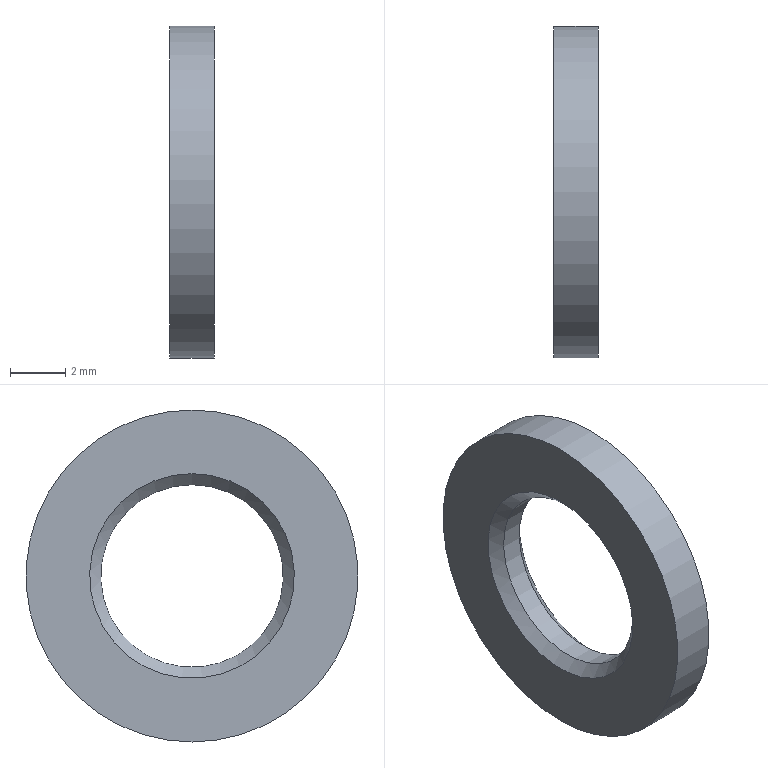Component | NX | WASHER_M6 | 1 solid | 6 faces | box 1.6 x 12 x 12 mm | volume 123 mm3 | cylinder 2 | plane 2 | cone 2 | commonest cylinder face diameters 12 x1 6.6 x1
STEP:
#1=CARTESIAN_POINT('',(0.,0.,0.));
#2=DIRECTION('',(0.,0.,1.));
#3=DIRECTION('',(1.,0.,0.));
#4=AXIS2_PLACEMENT_3D('',#1,#2,#3);
#5=CARTESIAN_POINT('',(10.307,66.5,-80.));
#6=VERTEX_POINT('',#5);
#7=CARTESIAN_POINT('',(10.307,66.5,-74.));
#8=DIRECTION('',(-1.,0.,0.));
#9=DIRECTION('',(0.,0.,-1.));
#10=AXIS2_PLACEMENT_3D('',#7,#8,#9);
#11=CIRCLE('',#10,6.);
#12=CARTESIAN_POINT('',(10.307,66.5,-74.));
#13=DIRECTION('',(-1.,0.,0.));
#14=DIRECTION('',(0.,0.,1.));
#15=AXIS2_PLACEMENT_3D('',#12,#13,#14);
#16=CYLINDRICAL_SURFACE('',#15,6.);
#17=CARTESIAN_POINT('',(3.142,0.));
#18=DIRECTION('',(1.,0.));
#19=VECTOR('',#18,1.);
#20=LINE('',#17,#19);
#21=(GEOMETRIC_REPRESENTATION_CONTEXT(2)PARAMETRIC_REPRESENTATION_CONTEXT()REPRESENTATION_CONTEXT('',''));
#22=DEFINITIONAL_REPRESENTATION('',(#20),#21);
#23=PCURVE('',#16,#22);
#24=CARTESIAN_POINT('',(10.307,66.5,-74.));
#25=DIRECTION('',(-1.,0.,0.));
#26=DIRECTION('',(0.,0.,1.));
#27=AXIS2_PLACEMENT_3D('',#24,#25,#26);
#28=PLANE('',#27);
#29=CARTESIAN_POINT('',(0.,0.));
#30=DIRECTION('',(-1.,0.));
#31=AXIS2_PLACEMENT_2D('',#29,#30);
#32=CIRCLE('',#31,6.);
#33=(GEOMETRIC_REPRESENTATION_CONTEXT(2)PARAMETRIC_REPRESENTATION_CONTEXT()REPRESENTATION_CONTEXT('',''));
#34=DEFINITIONAL_REPRESENTATION('',(#32),#33);
#35=PCURVE('',#28,#34);
#36=SURFACE_CURVE('',#11,(#23,#35),.PCURVE_S1.);
#37=EDGE_CURVE('',#6,#6,#36,.T.);
#38=ORIENTED_EDGE('',*,*,#37,.T.);
#39=CARTESIAN_POINT('',(8.707,66.5,-80.));
#40=VERTEX_POINT('',#39);
#41=CARTESIAN_POINT('',(10.307,66.5,-80.));
#42=CARTESIAN_POINT('',(8.707,66.5,-80.));
#43=B_SPLINE_CURVE_WITH_KNOTS('',1,(#41,#42),.UNSPECIFIED.,.F.,.F.,(2,2),(0.,1.6),.PIECEWISE_BEZIER_KNOTS.);
#44=CARTESIAN_POINT('',(9.425,0.));
#45=DIRECTION('',(0.,1.));
#46=VECTOR('',#45,1.);
#47=LINE('',#44,#46);
#48=(GEOMETRIC_REPRESENTATION_CONTEXT(2)PARAMETRIC_REPRESENTATION_CONTEXT()REPRESENTATION_CONTEXT('',''));
#49=DEFINITIONAL_REPRESENTATION('',(#47),#48);
#50=PCURVE('',#16,#49);
#51=CARTESIAN_POINT('',(3.142,0.));
#52=DIRECTION('',(0.,1.));
#53=VECTOR('',#52,1.);
#54=LINE('',#51,#53);
#55=(GEOMETRIC_REPRESENTATION_CONTEXT(2)PARAMETRIC_REPRESENTATION_CONTEXT()REPRESENTATION_CONTEXT('',''));
#56=DEFINITIONAL_REPRESENTATION('',(#54),#55);
#57=PCURVE('',#16,#56);
#58=SEAM_CURVE('',#43,(#50,#57),.PCURVE_S1.);
#59=EDGE_CURVE('',#6,#40,#58,.T.);
#60=ORIENTED_EDGE('',*,*,#59,.T.);
#61=CARTESIAN_POINT('',(8.707,66.5,-74.));
#62=DIRECTION('',(-1.,0.,0.));
#63=DIRECTION('',(0.,0.,-1.));
#64=AXIS2_PLACEMENT_3D('',#61,#62,#63);
#65=CIRCLE('',#64,6.);
#66=CARTESIAN_POINT('',(3.142,1.6));
#67=DIRECTION('',(1.,0.));
#68=VECTOR('',#67,1.);
#69=LINE('',#66,#68);
#70=(GEOMETRIC_REPRESENTATION_CONTEXT(2)PARAMETRIC_REPRESENTATION_CONTEXT()REPRESENTATION_CONTEXT('',''));
#71=DEFINITIONAL_REPRESENTATION('',(#69),#70);
#72=PCURVE('',#16,#71);
#73=CARTESIAN_POINT('',(8.707,66.5,-74.));
#74=DIRECTION('',(-1.,0.,0.));
#75=DIRECTION('',(0.,0.,1.));
#76=AXIS2_PLACEMENT_3D('',#73,#74,#75);
#77=PLANE('',#76);
#78=CARTESIAN_POINT('',(0.,0.));
#79=DIRECTION('',(-1.,0.));
#80=AXIS2_PLACEMENT_2D('',#78,#79);
#81=CIRCLE('',#80,6.);
#82=(GEOMETRIC_REPRESENTATION_CONTEXT(2)PARAMETRIC_REPRESENTATION_CONTEXT()REPRESENTATION_CONTEXT('',''));
#83=DEFINITIONAL_REPRESENTATION('',(#81),#82);
#84=PCURVE('',#77,#83);
#85=SURFACE_CURVE('',#65,(#72,#84),.PCURVE_S1.);
#86=EDGE_CURVE('',#40,#40,#85,.T.);
#87=ORIENTED_EDGE('',*,*,#86,.F.);
#88=ORIENTED_EDGE('',*,*,#59,.F.);
#89=EDGE_LOOP('',(#38,#60,#87,#88));
#90=FACE_BOUND('',#89,.T.);
#91=ADVANCED_FACE('',(#90),#16,.T.);
#92=CARTESIAN_POINT('',(9.907,66.5,-70.7));
#93=VERTEX_POINT('',#92);
#94=CARTESIAN_POINT('',(9.907,66.5,-74.));
#95=DIRECTION('',(1.,0.,0.));
#96=DIRECTION('',(0.,0.,1.));
#97=AXIS2_PLACEMENT_3D('',#94,#95,#96);
#98=CIRCLE('',#97,3.3);
#99=CARTESIAN_POINT('',(10.307,66.5,-74.));
#100=DIRECTION('',(-1.,0.,0.));
#101=DIRECTION('',(0.,0.,1.));
#102=AXIS2_PLACEMENT_3D('',#99,#100,#101);
#103=CYLINDRICAL_SURFACE('',#102,3.3);
#104=CARTESIAN_POINT('',(6.283,0.4));
#105=DIRECTION('',(-1.,0.));
#106=VECTOR('',#105,1.);
#107=LINE('',#104,#106);
#108=(GEOMETRIC_REPRESENTATION_CONTEXT(2)PARAMETRIC_REPRESENTATION_CONTEXT()REPRESENTATION_CONTEXT('',''));
#109=DEFINITIONAL_REPRESENTATION('',(#107),#108);
#110=PCURVE('',#103,#109);
#111=CARTESIAN_POINT('',(10.307,66.5,-74.));
#112=DIRECTION('',(1.,0.,0.));
#113=DIRECTION('',(0.,0.,-1.));
#114=AXIS2_PLACEMENT_3D('',#111,#112,#113);
#115=CONICAL_SURFACE('',#114,3.7,0.7854);
#116=CARTESIAN_POINT('',(3.142,-0.4));
#117=DIRECTION('',(1.,0.));
#118=VECTOR('',#117,1.);
#119=LINE('',#116,#118);
#120=(GEOMETRIC_REPRESENTATION_CONTEXT(2)PARAMETRIC_REPRESENTATION_CONTEXT()REPRESENTATION_CONTEXT('',''));
#121=DEFINITIONAL_REPRESENTATION('',(#119),#120);
#122=PCURVE('',#115,#121);
#123=SURFACE_CURVE('',#98,(#110,#122),.PCURVE_S1.);
#124=EDGE_CURVE('',#93,#93,#123,.T.);
#125=ORIENTED_EDGE('',*,*,#124,.F.);
#126=CARTESIAN_POINT('',(9.107,66.5,-70.7));
#127=VERTEX_POINT('',#126);
#128=CARTESIAN_POINT('',(9.907,66.5,-70.7));
#129=CARTESIAN_POINT('',(9.107,66.5,-70.7));
#130=B_SPLINE_CURVE_WITH_KNOTS('',1,(#128,#129),.UNSPECIFIED.,.F.,.F.,(2,2),(0.4,1.2),.PIECEWISE_BEZIER_KNOTS.);
#131=CARTESIAN_POINT('',(6.283,0.));
#132=DIRECTION('',(0.,1.));
#133=VECTOR('',#132,1.);
#134=LINE('',#131,#133);
#135=(GEOMETRIC_REPRESENTATION_CONTEXT(2)PARAMETRIC_REPRESENTATION_CONTEXT()REPRESENTATION_CONTEXT('',''));
#136=DEFINITIONAL_REPRESENTATION('',(#134),#135);
#137=PCURVE('',#103,#136);
#138=CARTESIAN_POINT('',(0.,0.));
#139=DIRECTION('',(0.,1.));
#140=VECTOR('',#139,1.);
#141=LINE('',#138,#140);
#142=(GEOMETRIC_REPRESENTATION_CONTEXT(2)PARAMETRIC_REPRESENTATION_CONTEXT()REPRESENTATION_CONTEXT('',''));
#143=DEFINITIONAL_REPRESENTATION('',(#141),#142);
#144=PCURVE('',#103,#143);
#145=SEAM_CURVE('',#130,(#137,#144),.PCURVE_S1.);
#146=EDGE_CURVE('',#93,#127,#145,.T.);
#147=ORIENTED_EDGE('',*,*,#146,.T.);
#148=CARTESIAN_POINT('',(9.107,66.5,-74.));
#149=DIRECTION('',(-1.,0.,0.));
#150=DIRECTION('',(0.,0.,1.));
#151=AXIS2_PLACEMENT_3D('',#148,#149,#150);
#152=CIRCLE('',#151,3.3);
#153=CARTESIAN_POINT('',(0.,1.2));
#154=DIRECTION('',(1.,0.));
#155=VECTOR('',#154,1.);
#156=LINE('',#153,#155);
#157=(GEOMETRIC_REPRESENTATION_CONTEXT(2)PARAMETRIC_REPRESENTATION_CONTEXT()REPRESENTATION_CONTEXT('',''));
#158=DEFINITIONAL_REPRESENTATION('',(#156),#157);
#159=PCURVE('',#103,#158);
#160=CARTESIAN_POINT('',(9.107,66.5,-74.));
#161=DIRECTION('',(-1.,0.,0.));
#162=DIRECTION('',(0.,0.,1.));
#163=AXIS2_PLACEMENT_3D('',#160,#161,#162);
#164=CONICAL_SURFACE('',#163,3.3,0.7854);
#165=CARTESIAN_POINT('',(0.,-0.));
#166=DIRECTION('',(1.,0.));
#167=VECTOR('',#166,1.);
#168=LINE('',#165,#167);
#169=(GEOMETRIC_REPRESENTATION_CONTEXT(2)PARAMETRIC_REPRESENTATION_CONTEXT()REPRESENTATION_CONTEXT('',''));
#170=DEFINITIONAL_REPRESENTATION('',(#168),#169);
#171=PCURVE('',#164,#170);
#172=SURFACE_CURVE('',#152,(#159,#171),.PCURVE_S1.);
#173=EDGE_CURVE('',#127,#127,#172,.T.);
#174=ORIENTED_EDGE('',*,*,#173,.F.);
#175=ORIENTED_EDGE('',*,*,#146,.F.);
#176=EDGE_LOOP('',(#125,#147,#174,#175));
#177=FACE_BOUND('',#176,.F.);
#178=ADVANCED_FACE('',(#177),#103,.F.);
#179=CARTESIAN_POINT('',(10.307,66.5,-70.3));
#180=VERTEX_POINT('',#179);
#181=CARTESIAN_POINT('',(10.307,66.5,-74.));
#182=DIRECTION('',(-1.,0.,0.));
#183=DIRECTION('',(0.,0.,1.));
#184=AXIS2_PLACEMENT_3D('',#181,#182,#183);
#185=CIRCLE('',#184,3.7);
#186=CARTESIAN_POINT('',(0.,0.));
#187=DIRECTION('',(1.,0.));
#188=AXIS2_PLACEMENT_2D('',#186,#187);
#189=CIRCLE('',#188,3.7);
#190=(GEOMETRIC_REPRESENTATION_CONTEXT(2)PARAMETRIC_REPRESENTATION_CONTEXT()REPRESENTATION_CONTEXT('',''));
#191=DEFINITIONAL_REPRESENTATION('',(#189),#190);
#192=PCURVE('',#28,#191);
#193=CARTESIAN_POINT('',(9.425,-0.));
#194=DIRECTION('',(-1.,0.));
#195=VECTOR('',#194,1.);
#196=LINE('',#193,#195);
#197=(GEOMETRIC_REPRESENTATION_CONTEXT(2)PARAMETRIC_REPRESENTATION_CONTEXT()REPRESENTATION_CONTEXT('',''));
#198=DEFINITIONAL_REPRESENTATION('',(#196),#197);
#199=PCURVE('',#115,#198);
#200=SURFACE_CURVE('',#185,(#192,#199),.PCURVE_S1.);
#201=EDGE_CURVE('',#180,#180,#200,.T.);
#202=ORIENTED_EDGE('',*,*,#201,.T.);
#203=EDGE_LOOP('',(#202));
#204=FACE_BOUND('',#203,.T.);
#205=ORIENTED_EDGE('',*,*,#37,.F.);
#206=EDGE_LOOP('',(#205));
#207=FACE_BOUND('',#206,.T.);
#208=ADVANCED_FACE('',(#204,#207),#28,.F.);
#209=CARTESIAN_POINT('',(8.707,66.5,-70.3));
#210=VERTEX_POINT('',#209);
#211=CARTESIAN_POINT('',(8.707,66.5,-74.));
#212=DIRECTION('',(1.,0.,0.));
#213=DIRECTION('',(0.,0.,1.));
#214=AXIS2_PLACEMENT_3D('',#211,#212,#213);
#215=CIRCLE('',#214,3.7);
#216=CARTESIAN_POINT('',(3.7,0.));
#217=CARTESIAN_POINT('',(3.7,-6.409));
#218=CARTESIAN_POINT('',(-1.85,-3.204));
#219=CARTESIAN_POINT('',(-7.4,-0.));
#220=CARTESIAN_POINT('',(-1.85,3.204));
#221=CARTESIAN_POINT('',(3.7,6.409));
#222=CARTESIAN_POINT('',(3.7,0.));
#223=(BOUNDED_CURVE()B_SPLINE_CURVE(2,(#216,#217,#218,#219,#220,#221,#222),.UNSPECIFIED.,.T.,.F.)B_SPLINE_CURVE_WITH_KNOTS((1,2,2,2,2,1),(-2.094,0.,2.094,4.189,6.283,8.378),.UNSPECIFIED.)CURVE()GEOMETRIC_REPRESENTATION_ITEM()RATIONAL_B_SPLINE_CURVE((1.,0.5,1.,0.5,1.,0.5,1.))REPRESENTATION_ITEM(''));
#224=(GEOMETRIC_REPRESENTATION_CONTEXT(2)PARAMETRIC_REPRESENTATION_CONTEXT()REPRESENTATION_CONTEXT('',''));
#225=DEFINITIONAL_REPRESENTATION('',(#223),#224);
#226=PCURVE('',#77,#225);
#227=CARTESIAN_POINT('',(6.283,0.4));
#228=DIRECTION('',(-1.,0.));
#229=VECTOR('',#228,1.);
#230=LINE('',#227,#229);
#231=(GEOMETRIC_REPRESENTATION_CONTEXT(2)PARAMETRIC_REPRESENTATION_CONTEXT()REPRESENTATION_CONTEXT('',''));
#232=DEFINITIONAL_REPRESENTATION('',(#230),#231);
#233=PCURVE('',#164,#232);
#234=SURFACE_CURVE('',#215,(#226,#233),.PCURVE_S1.);
#235=EDGE_CURVE('',#210,#210,#234,.T.);
#236=ORIENTED_EDGE('',*,*,#235,.T.);
#237=EDGE_LOOP('',(#236));
#238=FACE_BOUND('',#237,.T.);
#239=ORIENTED_EDGE('',*,*,#86,.T.);
#240=EDGE_LOOP('',(#239));
#241=FACE_BOUND('',#240,.T.);
#242=ADVANCED_FACE('',(#238,#241),#77,.T.);
#243=ORIENTED_EDGE('',*,*,#124,.T.);
#244=CARTESIAN_POINT('',(9.907,66.5,-70.7));
#245=CARTESIAN_POINT('',(10.307,66.5,-70.3));
#246=B_SPLINE_CURVE_WITH_KNOTS('',1,(#244,#245),.UNSPECIFIED.,.F.,.F.,(2,2),(-0.5657,-0.),.PIECEWISE_BEZIER_KNOTS.);
#247=CARTESIAN_POINT('',(9.425,0.));
#248=DIRECTION('',(0.,1.));
#249=VECTOR('',#248,1.);
#250=LINE('',#247,#249);
#251=(GEOMETRIC_REPRESENTATION_CONTEXT(2)PARAMETRIC_REPRESENTATION_CONTEXT()REPRESENTATION_CONTEXT('',''));
#252=DEFINITIONAL_REPRESENTATION('',(#250),#251);
#253=PCURVE('',#115,#252);
#254=CARTESIAN_POINT('',(3.142,0.));
#255=DIRECTION('',(0.,1.));
#256=VECTOR('',#255,1.);
#257=LINE('',#254,#256);
#258=(GEOMETRIC_REPRESENTATION_CONTEXT(2)PARAMETRIC_REPRESENTATION_CONTEXT()REPRESENTATION_CONTEXT('',''));
#259=DEFINITIONAL_REPRESENTATION('',(#257),#258);
#260=PCURVE('',#115,#259);
#261=SEAM_CURVE('',#246,(#253,#260),.PCURVE_S1.);
#262=EDGE_CURVE('',#93,#180,#261,.T.);
#263=ORIENTED_EDGE('',*,*,#262,.T.);
#264=ORIENTED_EDGE('',*,*,#201,.T.);
#265=ORIENTED_EDGE('',*,*,#262,.F.);
#266=EDGE_LOOP('',(#243,#263,#264,#265));
#267=FACE_BOUND('',#266,.F.);
#268=ADVANCED_FACE('',(#267),#115,.F.);
#269=ORIENTED_EDGE('',*,*,#235,.T.);
#270=CARTESIAN_POINT('',(9.107,66.5,-70.7));
#271=CARTESIAN_POINT('',(8.707,66.5,-70.3));
#272=B_SPLINE_CURVE_WITH_KNOTS('',1,(#270,#271),.UNSPECIFIED.,.F.,.F.,(2,2),(-0.,0.5657),.PIECEWISE_BEZIER_KNOTS.);
#273=CARTESIAN_POINT('',(0.,0.));
#274=DIRECTION('',(0.,1.));
#275=VECTOR('',#274,1.);
#276=LINE('',#273,#275);
#277=(GEOMETRIC_REPRESENTATION_CONTEXT(2)PARAMETRIC_REPRESENTATION_CONTEXT()REPRESENTATION_CONTEXT('',''));
#278=DEFINITIONAL_REPRESENTATION('',(#276),#277);
#279=PCURVE('',#164,#278);
#280=CARTESIAN_POINT('',(6.283,0.));
#281=DIRECTION('',(0.,1.));
#282=VECTOR('',#281,1.);
#283=LINE('',#280,#282);
#284=(GEOMETRIC_REPRESENTATION_CONTEXT(2)PARAMETRIC_REPRESENTATION_CONTEXT()REPRESENTATION_CONTEXT('',''));
#285=DEFINITIONAL_REPRESENTATION('',(#283),#284);
#286=PCURVE('',#164,#285);
#287=SEAM_CURVE('',#272,(#279,#286),.PCURVE_S1.);
#288=EDGE_CURVE('',#127,#210,#287,.T.);
#289=ORIENTED_EDGE('',*,*,#288,.F.);
#290=ORIENTED_EDGE('',*,*,#173,.T.);
#291=ORIENTED_EDGE('',*,*,#288,.T.);
#292=EDGE_LOOP('',(#269,#289,#290,#291));
#293=FACE_BOUND('',#292,.F.);
#294=ADVANCED_FACE('',(#293),#164,.F.);
#295=CLOSED_SHELL('',(#91,#178,#208,#242,#268,#294));
#296=MANIFOLD_SOLID_BREP('',#295);
#297=(LENGTH_UNIT()NAMED_UNIT(*)SI_UNIT(.MILLI.,.METRE.));
#298=UNCERTAINTY_MEASURE_WITH_UNIT(LENGTH_MEASURE(0.00001),#297,'','');
#299=(NAMED_UNIT(*)PLANE_ANGLE_UNIT()SI_UNIT($,.RADIAN.));
#300=(NAMED_UNIT(*)SI_UNIT($,.STERADIAN.)SOLID_ANGLE_UNIT());
#301=(GEOMETRIC_REPRESENTATION_CONTEXT(3)GLOBAL_UNCERTAINTY_ASSIGNED_CONTEXT((#298))GLOBAL_UNIT_ASSIGNED_CONTEXT((#297,#299,#300))REPRESENTATION_CONTEXT('',''));
#302=ADVANCED_BREP_SHAPE_REPRESENTATION('',(#4,#296),#301);